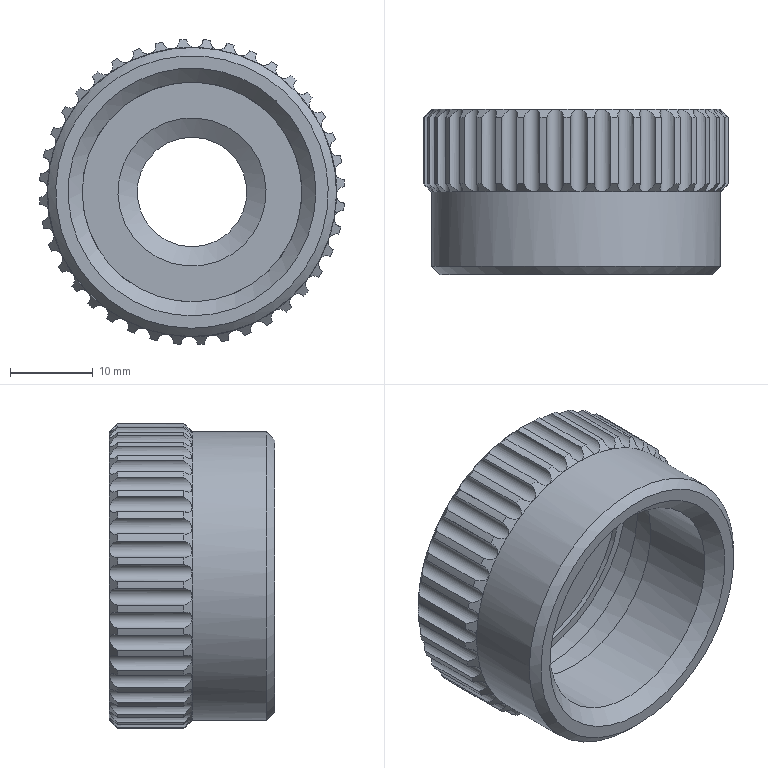Component | NX | 2 | 1 solid | 174 faces | volume 7487 mm3 | cylinder 85 | cone 83 | plane 6 | commonest cylinder face diameters 37 x40 2 x40 30 x2 35 x1 26.59 x1 32 x1